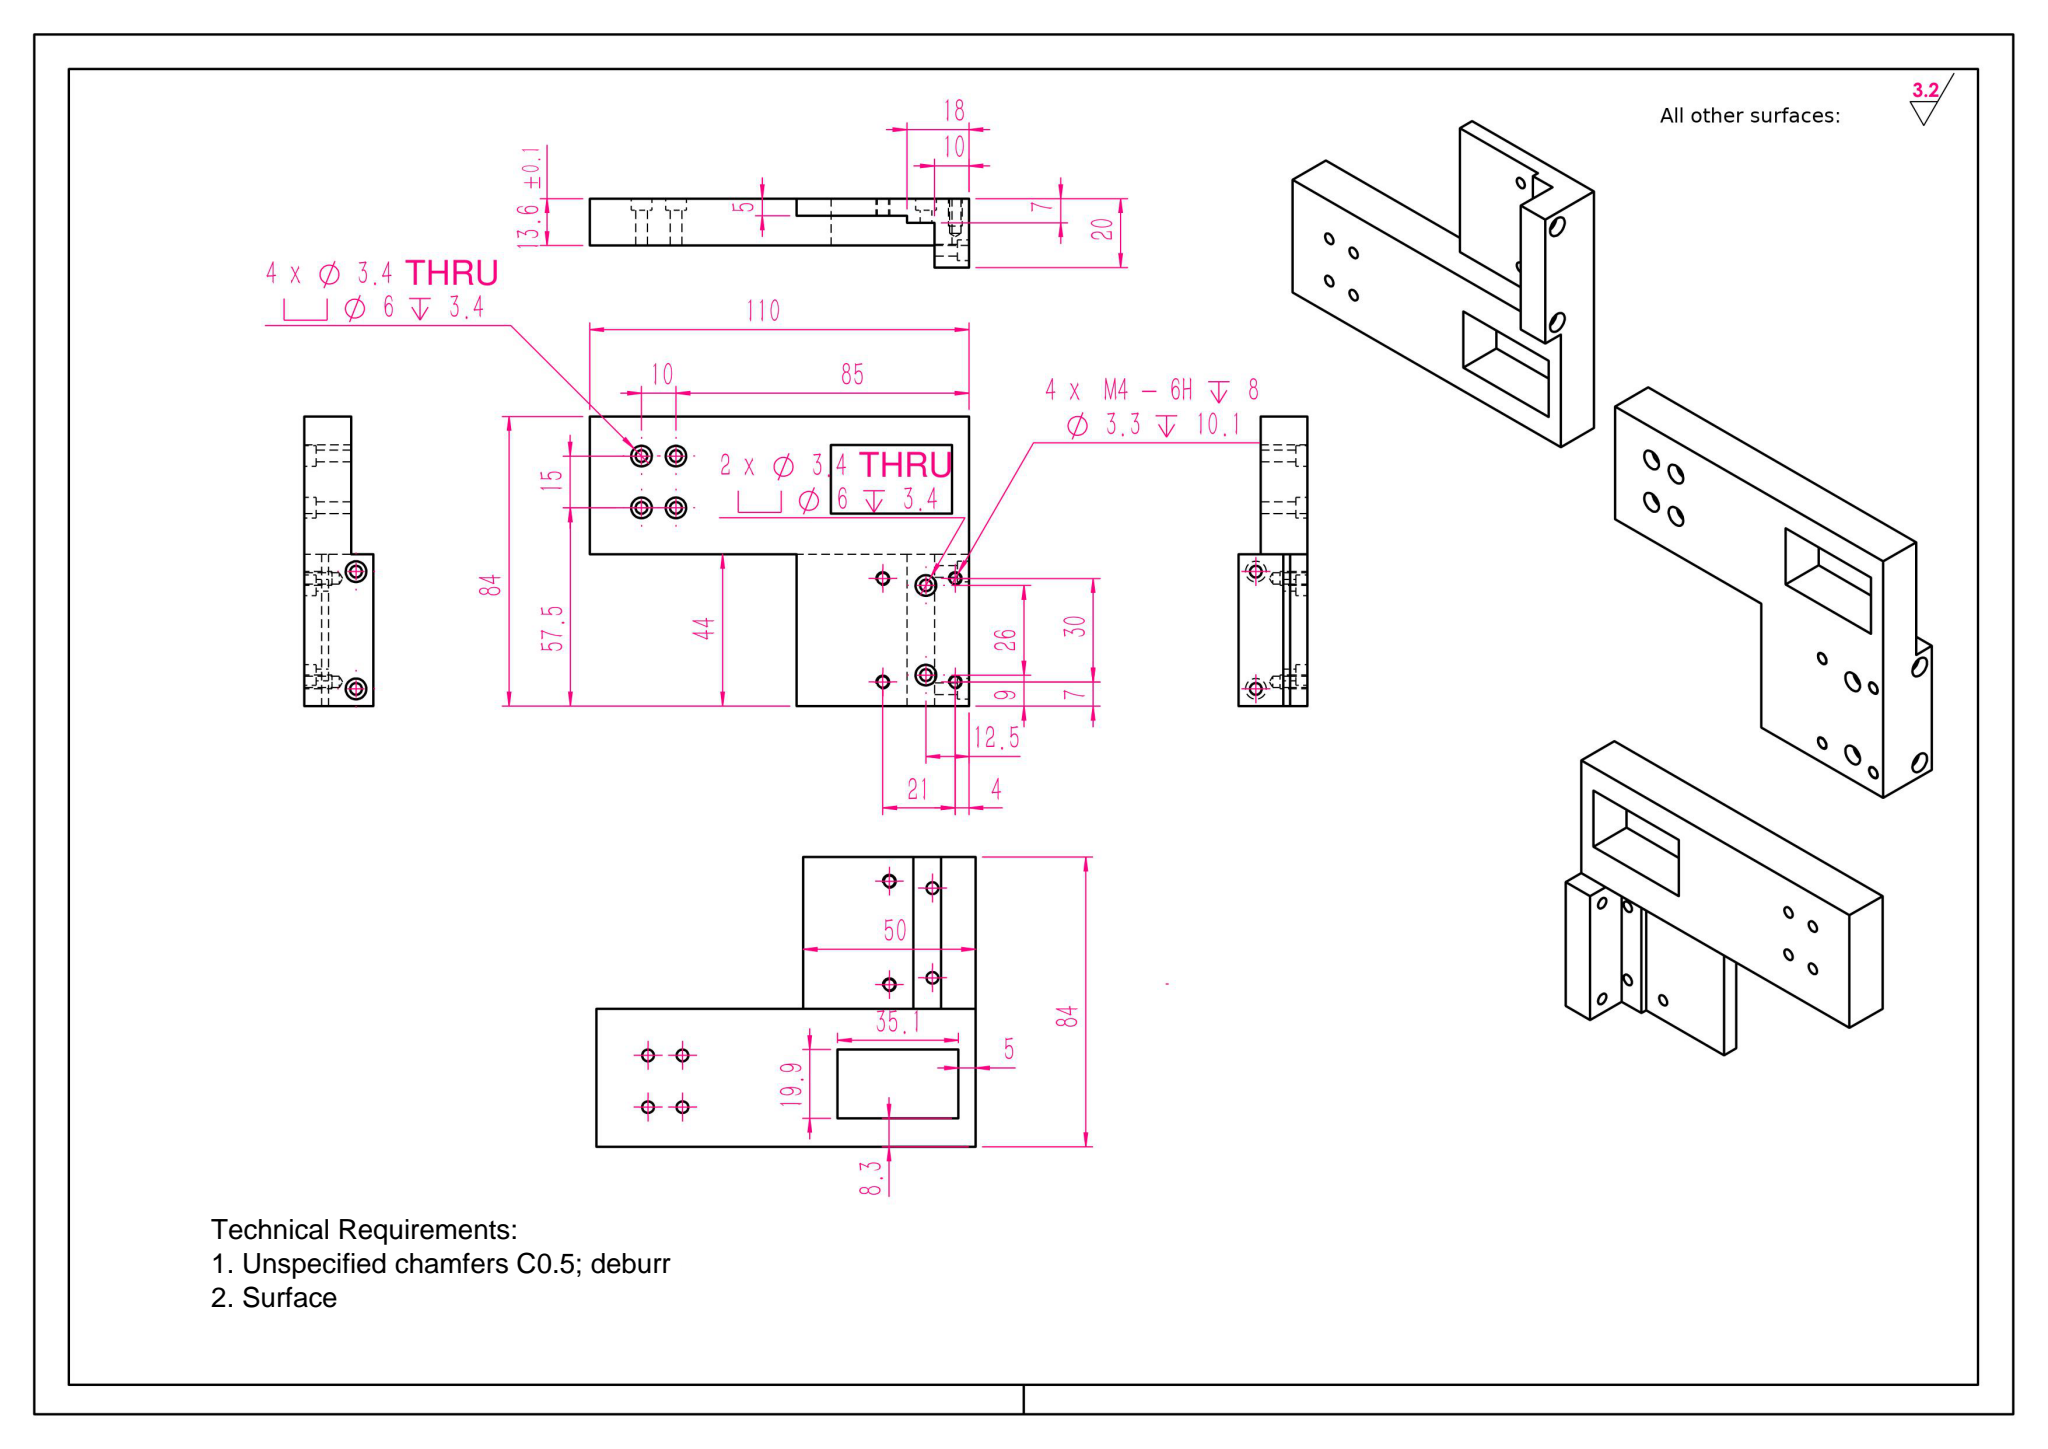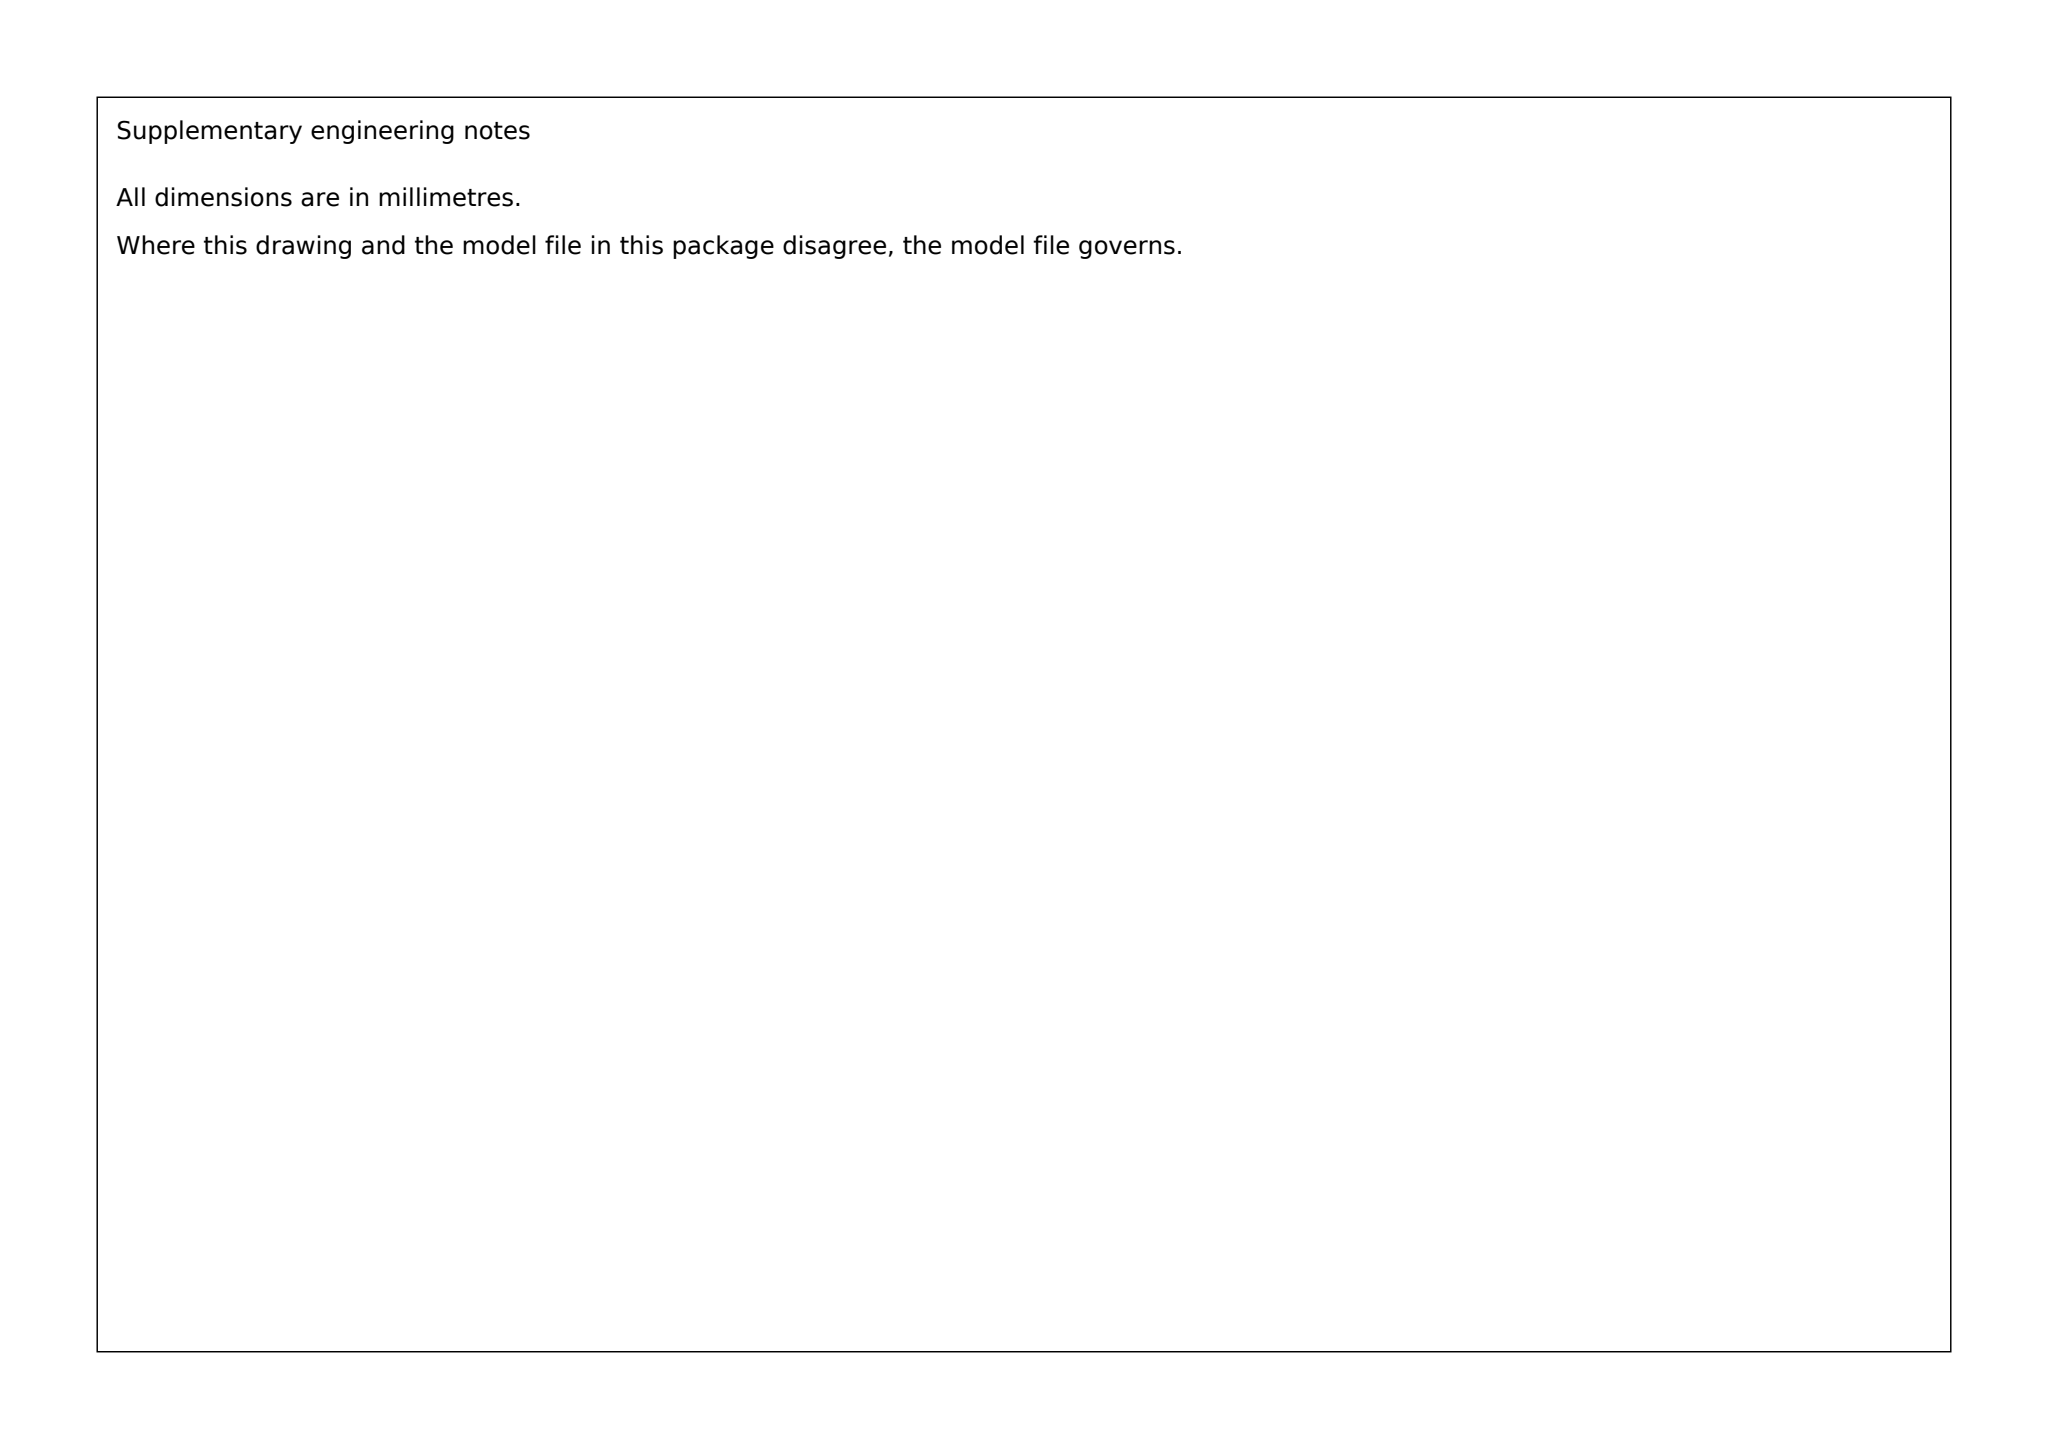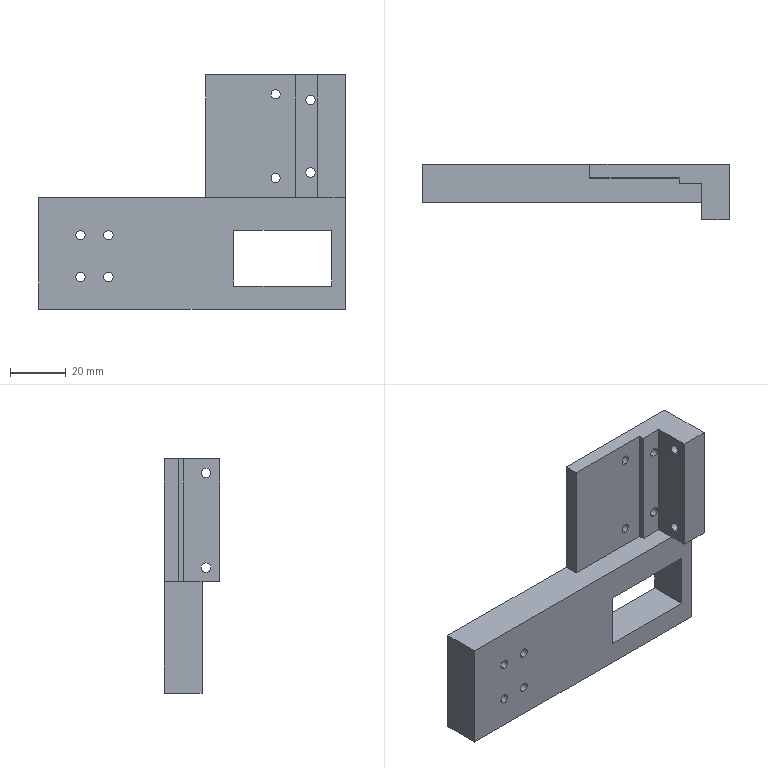Part | SolidWorks | mm | 1 solid | 70 faces | box 110 x 20 x 84 mm | volume 67047 mm3 | cylinder 40 | plane 26 | cone 4 | commonest cylinder face diameters 6 x16 3.4 x16 3.3 x8
build123d program:
from build123d import *

# Parameters (mm, degrees)
SKETCH1_W                                            = 50
SKETCH1_H                                            = 44
BOSS_EXTRUDE1_DEPTH                                  = 20
SKETCH2_W                                            = 40
SKETCH2_H                                            = 13
CUT_EXTRUDE1_DEPTH                                   = 55.415
SKETCH3_W                                            = 32
SKETCH3_H                                            = 2
CUT_EXTRUDE2_DEPTH                                   = 55.415
HOLE_SIZE_ACCORDING_TO_HEX_SOCKET_HEAD_C_D           = 3.4
HOLE_SIZE_ACCORDING_TO_HEX_SOCKET_HEAD_C_CBORE_D     = 6
HOLE_SIZE_ACCORDING_TO_HEX_SOCKET_HEAD_C_CBORE_DEPTH = 3.4
HOLE_SIZE_ACCORDING_TO_HEX_SOCKET_HE_2_D             = 3.4
HOLE_SIZE_ACCORDING_TO_HEX_SOCKET_HE_2_CBORE_D       = 6
HOLE_SIZE_ACCORDING_TO_HEX_SOCKET_HE_2_CBORE_DEPTH   = 3.4
M4_TAPPED_HOLE1_D                                    = 3.3
M4_TAPPED_HOLE1_DEPTH                                = 10.1
M4_TAPPED_HOLE1_TIP                                  = 0.9914
SKETCH13_W                                           = 110
SKETCH13_H                                           = 13.6
BOSS_EXTRUDE2_DEPTH                                  = 40
HOLE_SIZE_ACCORDING_TO_HEX_SOCKET_HE_3_D             = 3.4
HOLE_SIZE_ACCORDING_TO_HEX_SOCKET_HE_3_CBORE_D       = 6
HOLE_SIZE_ACCORDING_TO_HEX_SOCKET_HE_3_CBORE_DEPTH   = 3.4
SKETCH16_W                                           = 35.077
SKETCH16_H                                           = 19.932
CUT_EXTRUDE3_DEPTH                                   = 56


with BuildPart() as part:
    # Sketch1 → Boss-Extrude1 (new body)
    with BuildSketch(Plane(origin=(0, 0, 0), x_dir=(1, 0, 0), z_dir=(0, 1, 0))):
        Rectangle(SKETCH1_W, SKETCH1_H)
    extrude(amount=BOSS_EXTRUDE1_DEPTH)

    # Sketch2 → Cut-Extrude1 (cut, through all)
    with BuildSketch(Plane(origin=(0, 0, -22), x_dir=(-1, 0, 0), z_dir=(0, 0, -1))):
        with Locations((5, 6.5)):
            Rectangle(SKETCH2_W, SKETCH2_H)
    extrude(amount=-CUT_EXTRUDE1_DEPTH, mode=Mode.SUBTRACT)

    # Sketch3 → Cut-Extrude2 (cut, through all)
    with BuildSketch(Plane(origin=(0, 0, -22), x_dir=(-1, 0, 0), z_dir=(0, 0, -1))):
        with Locations((9, 14)):
            Rectangle(SKETCH3_W, SKETCH3_H)
    extrude(amount=-CUT_EXTRUDE2_DEPTH, mode=Mode.SUBTRACT)

    # Hole Size according to Hex Socket Head C (through all)
    with Locations(Plane(origin=(25, 0, 0), x_dir=(0, 0, -1), z_dir=(1, 0, 0))):
        with Locations((-17, 5), (17, 5)):
            CounterBoreHole(HOLE_SIZE_ACCORDING_TO_HEX_SOCKET_HEAD_C_D / 2, HOLE_SIZE_ACCORDING_TO_HEX_SOCKET_HEAD_C_CBORE_D / 2, HOLE_SIZE_ACCORDING_TO_HEX_SOCKET_HEAD_C_CBORE_DEPTH)

    # Hole Size according to Hex Socket He 2 (through all)
    with Locations(Plane(origin=(0, 20, 0), x_dir=(1, 0, 0), z_dir=(0, 1, 0))):
        with Locations((12.5, 13), (12.5, -13)):
            CounterBoreHole(HOLE_SIZE_ACCORDING_TO_HEX_SOCKET_HE_2_D / 2, HOLE_SIZE_ACCORDING_TO_HEX_SOCKET_HE_2_CBORE_D / 2, HOLE_SIZE_ACCORDING_TO_HEX_SOCKET_HE_2_CBORE_DEPTH)

    # M4 Tapped Hole1
    with Locations(Plane(origin=(0, 20, 0), x_dir=(1, 0, 0), z_dir=(0, 1, 0))):
        with Locations((0, 15), (0, -15), (21, 15), (21, -15)):
            Hole(M4_TAPPED_HOLE1_D / 2, depth=M4_TAPPED_HOLE1_DEPTH)
            with Locations((0, 0, -(M4_TAPPED_HOLE1_DEPTH + M4_TAPPED_HOLE1_TIP / 2))):  # 118° drill point
                Cone(0, M4_TAPPED_HOLE1_D / 2, M4_TAPPED_HOLE1_TIP, mode=Mode.SUBTRACT)

    # Sketch13 → Boss-Extrude2 (add)
    with BuildSketch(Plane(origin=(0, 0, -22), x_dir=(-1, 0, 0), z_dir=(0, 0, -1))):
        with Locations((30, 13.2)):
            Rectangle(SKETCH13_W, SKETCH13_H)
    extrude(amount=BOSS_EXTRUDE2_DEPTH)

    # Hole Size according to Hex Socket He 3 (through all)
    with Locations(Plane(origin=(0, 20, 0), x_dir=(1, 0, 0), z_dir=(0, 1, 0))):
        with Locations((-70, 50.5), (-70, 35.5), (-60, 35.5), (-60, 50.5)):
            CounterBoreHole(HOLE_SIZE_ACCORDING_TO_HEX_SOCKET_HE_3_D / 2, HOLE_SIZE_ACCORDING_TO_HEX_SOCKET_HE_3_CBORE_D / 2, HOLE_SIZE_ACCORDING_TO_HEX_SOCKET_HE_3_CBORE_DEPTH)

    # Sketch16 → Cut-Extrude3 (cut)
    with BuildSketch(Plane.XZ.offset(-6.4)):
        with Locations((2.51, -43.762)):
            Rectangle(SKETCH16_W, SKETCH16_H)
    extrude(amount=-CUT_EXTRUDE3_DEPTH, mode=Mode.SUBTRACT)


solid = part.part